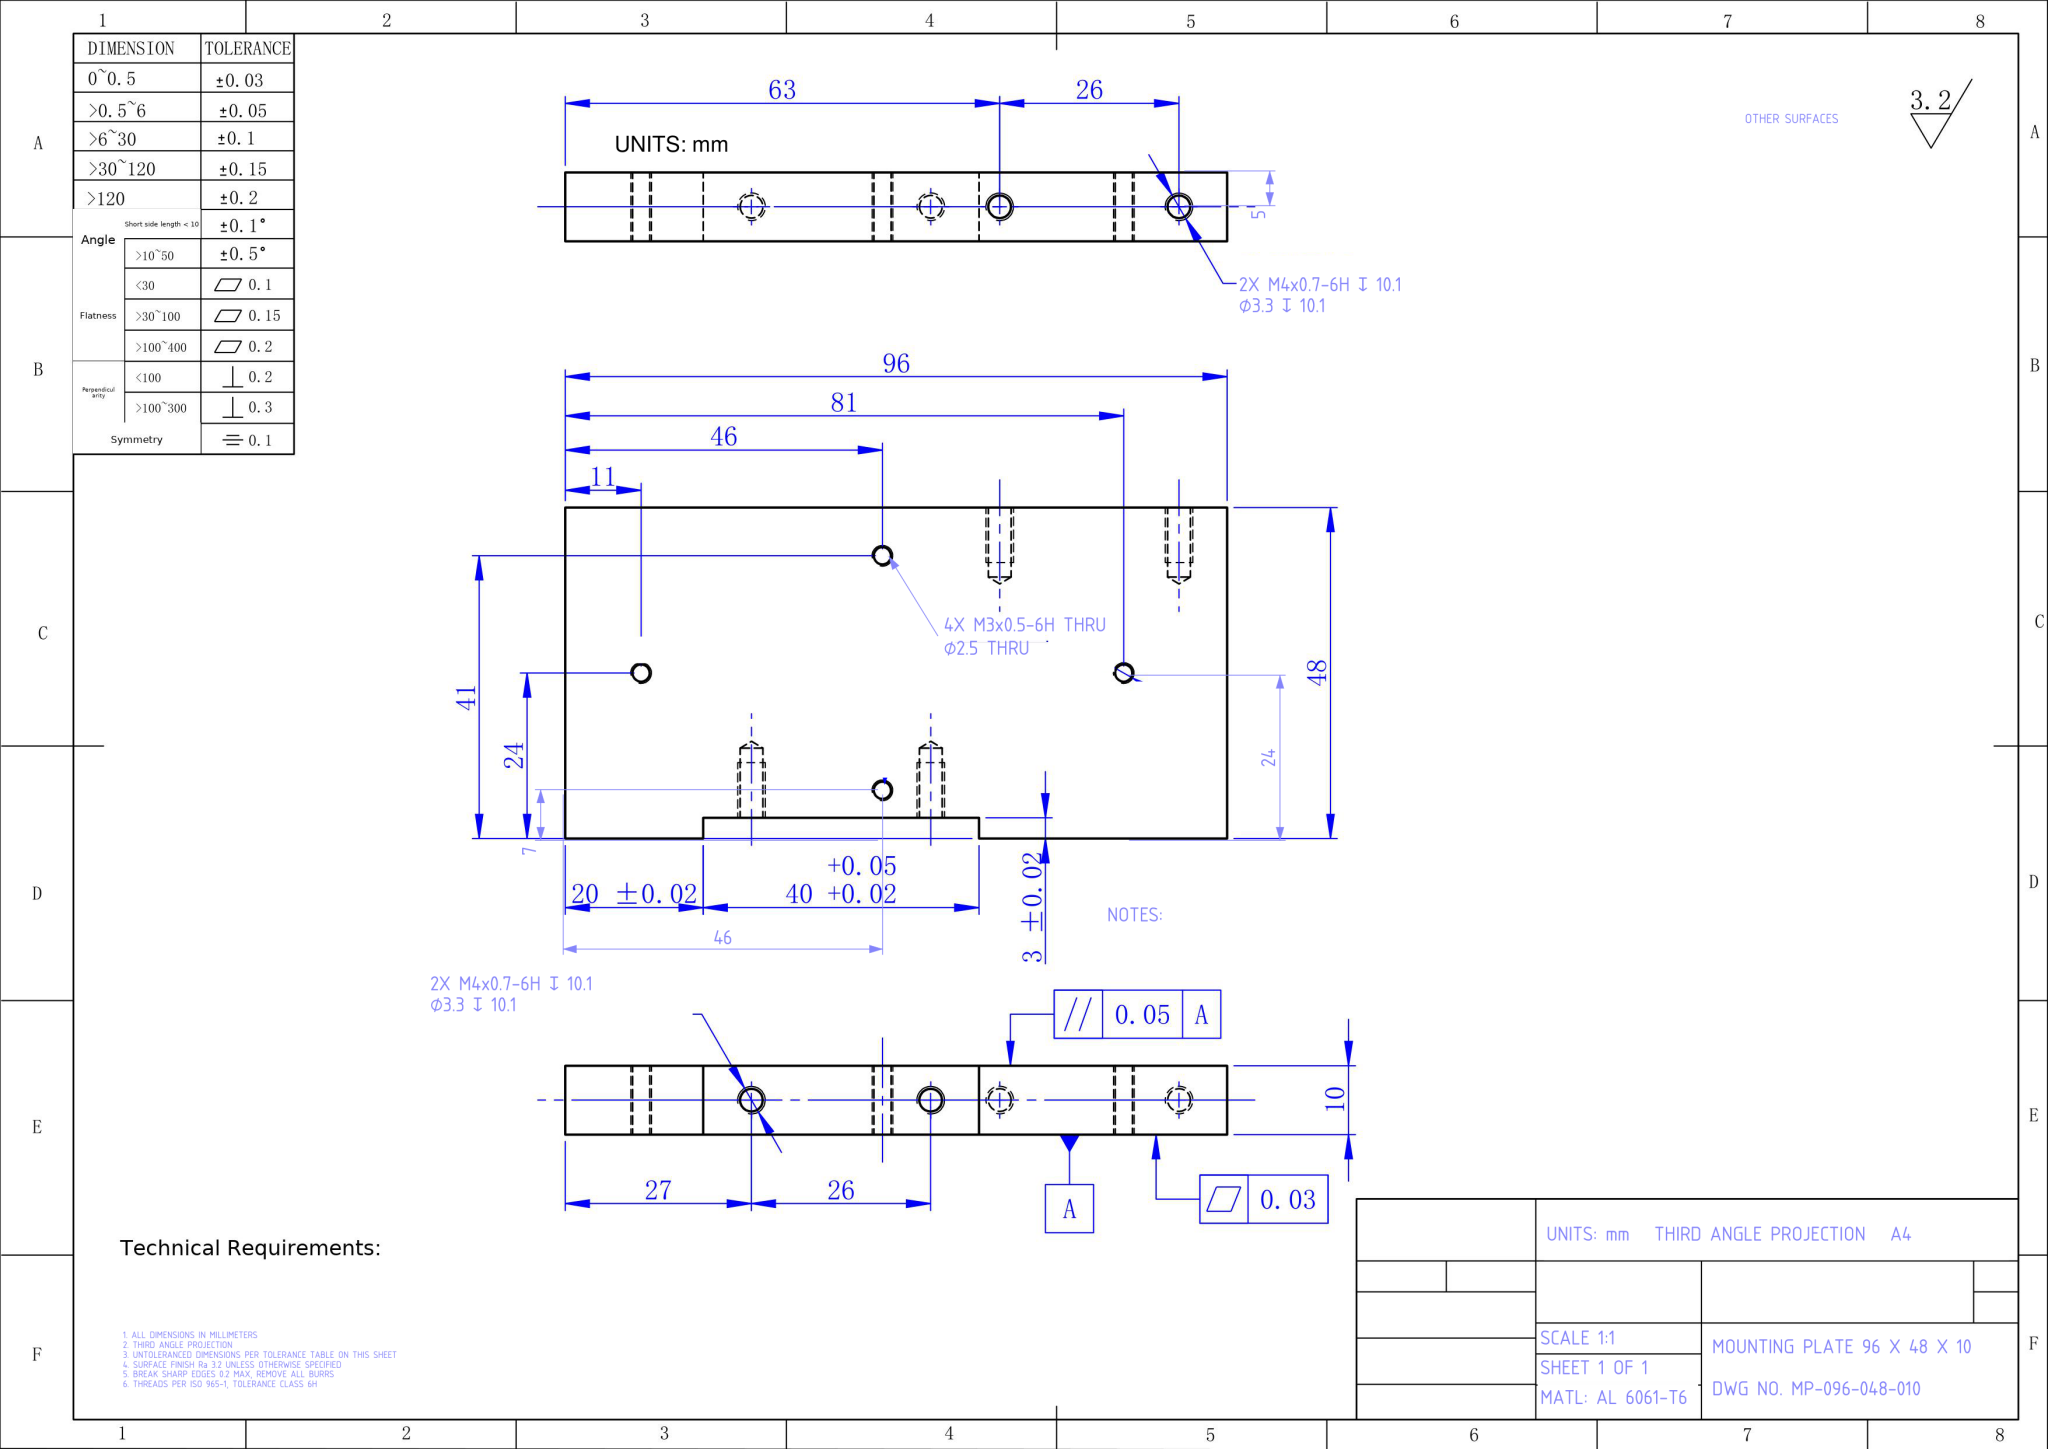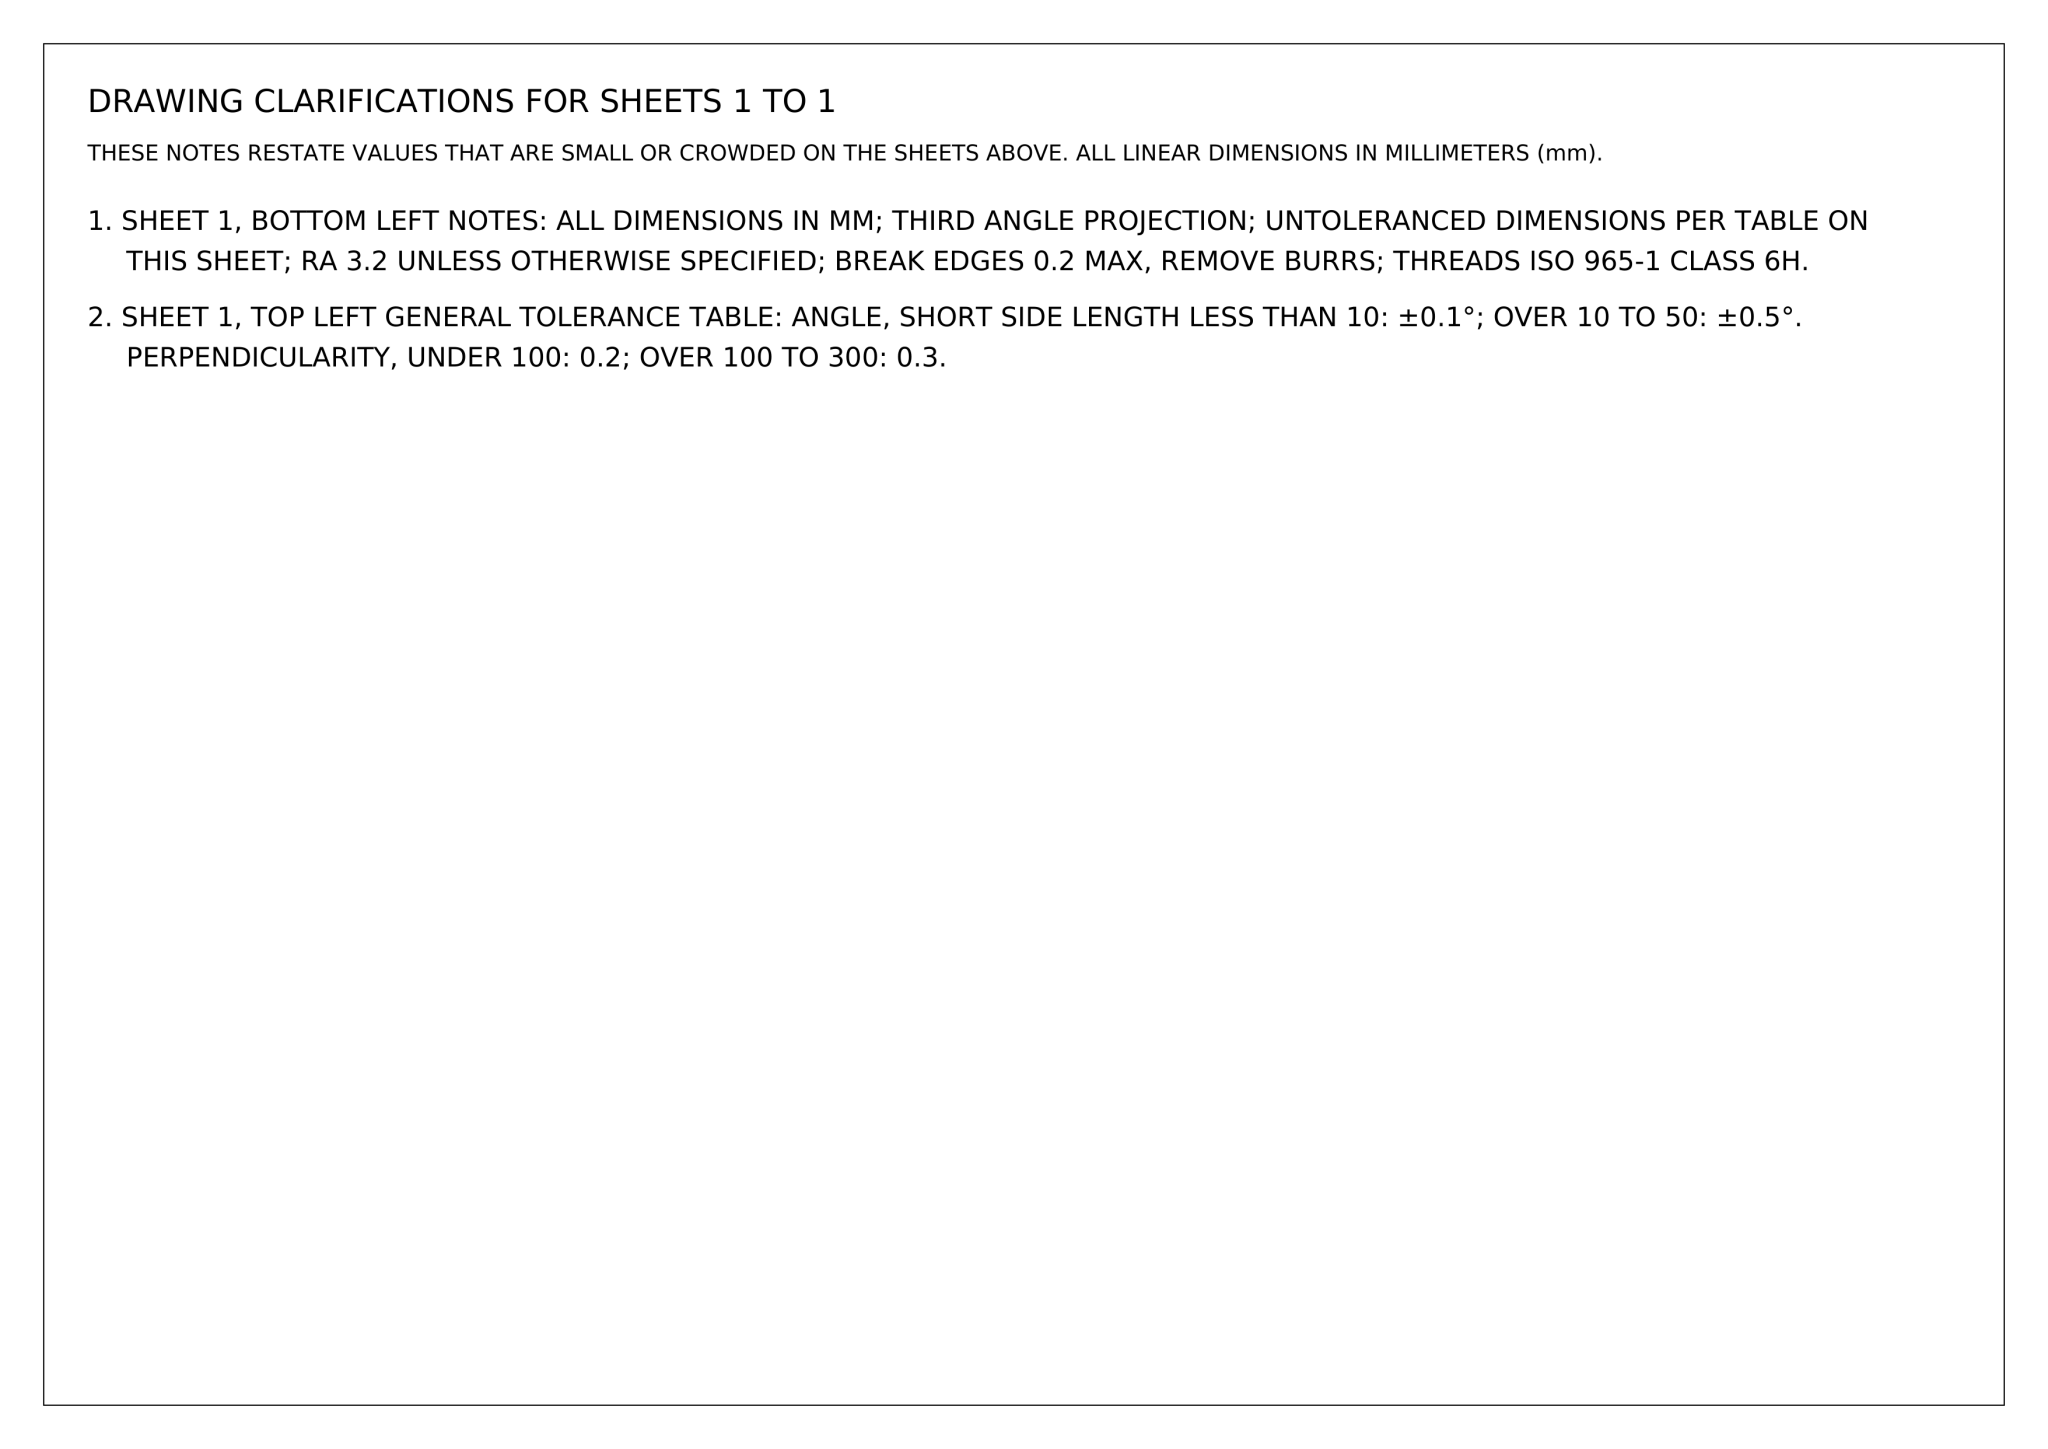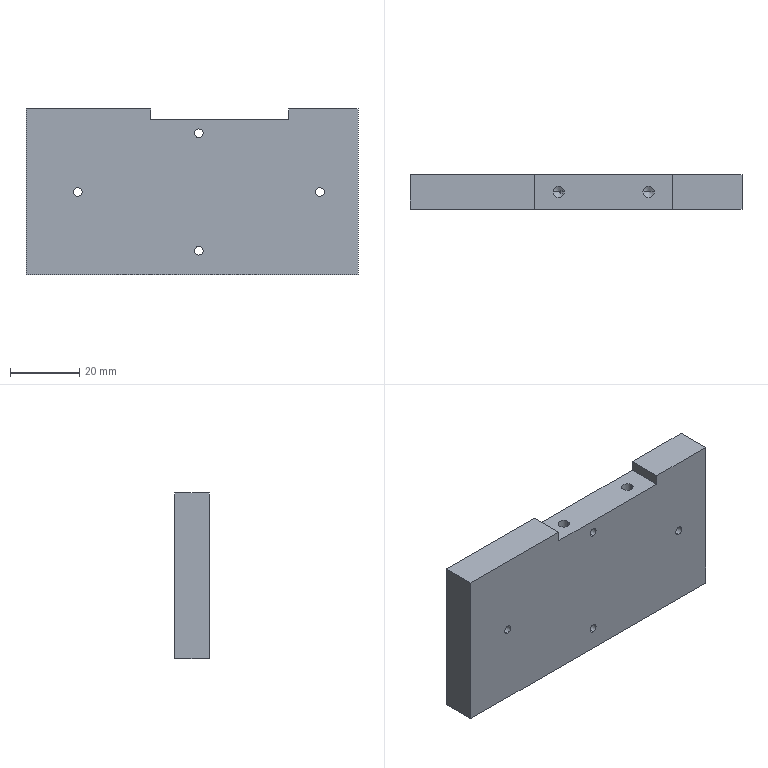Part | NX | mm | 1 solid | 34 faces | box 96 x 10 x 48 mm | volume 44327 mm3 | cylinder 16 | plane 10 | cone 8 | commonest cylinder face diameters 3.3 x8 2.5 x8